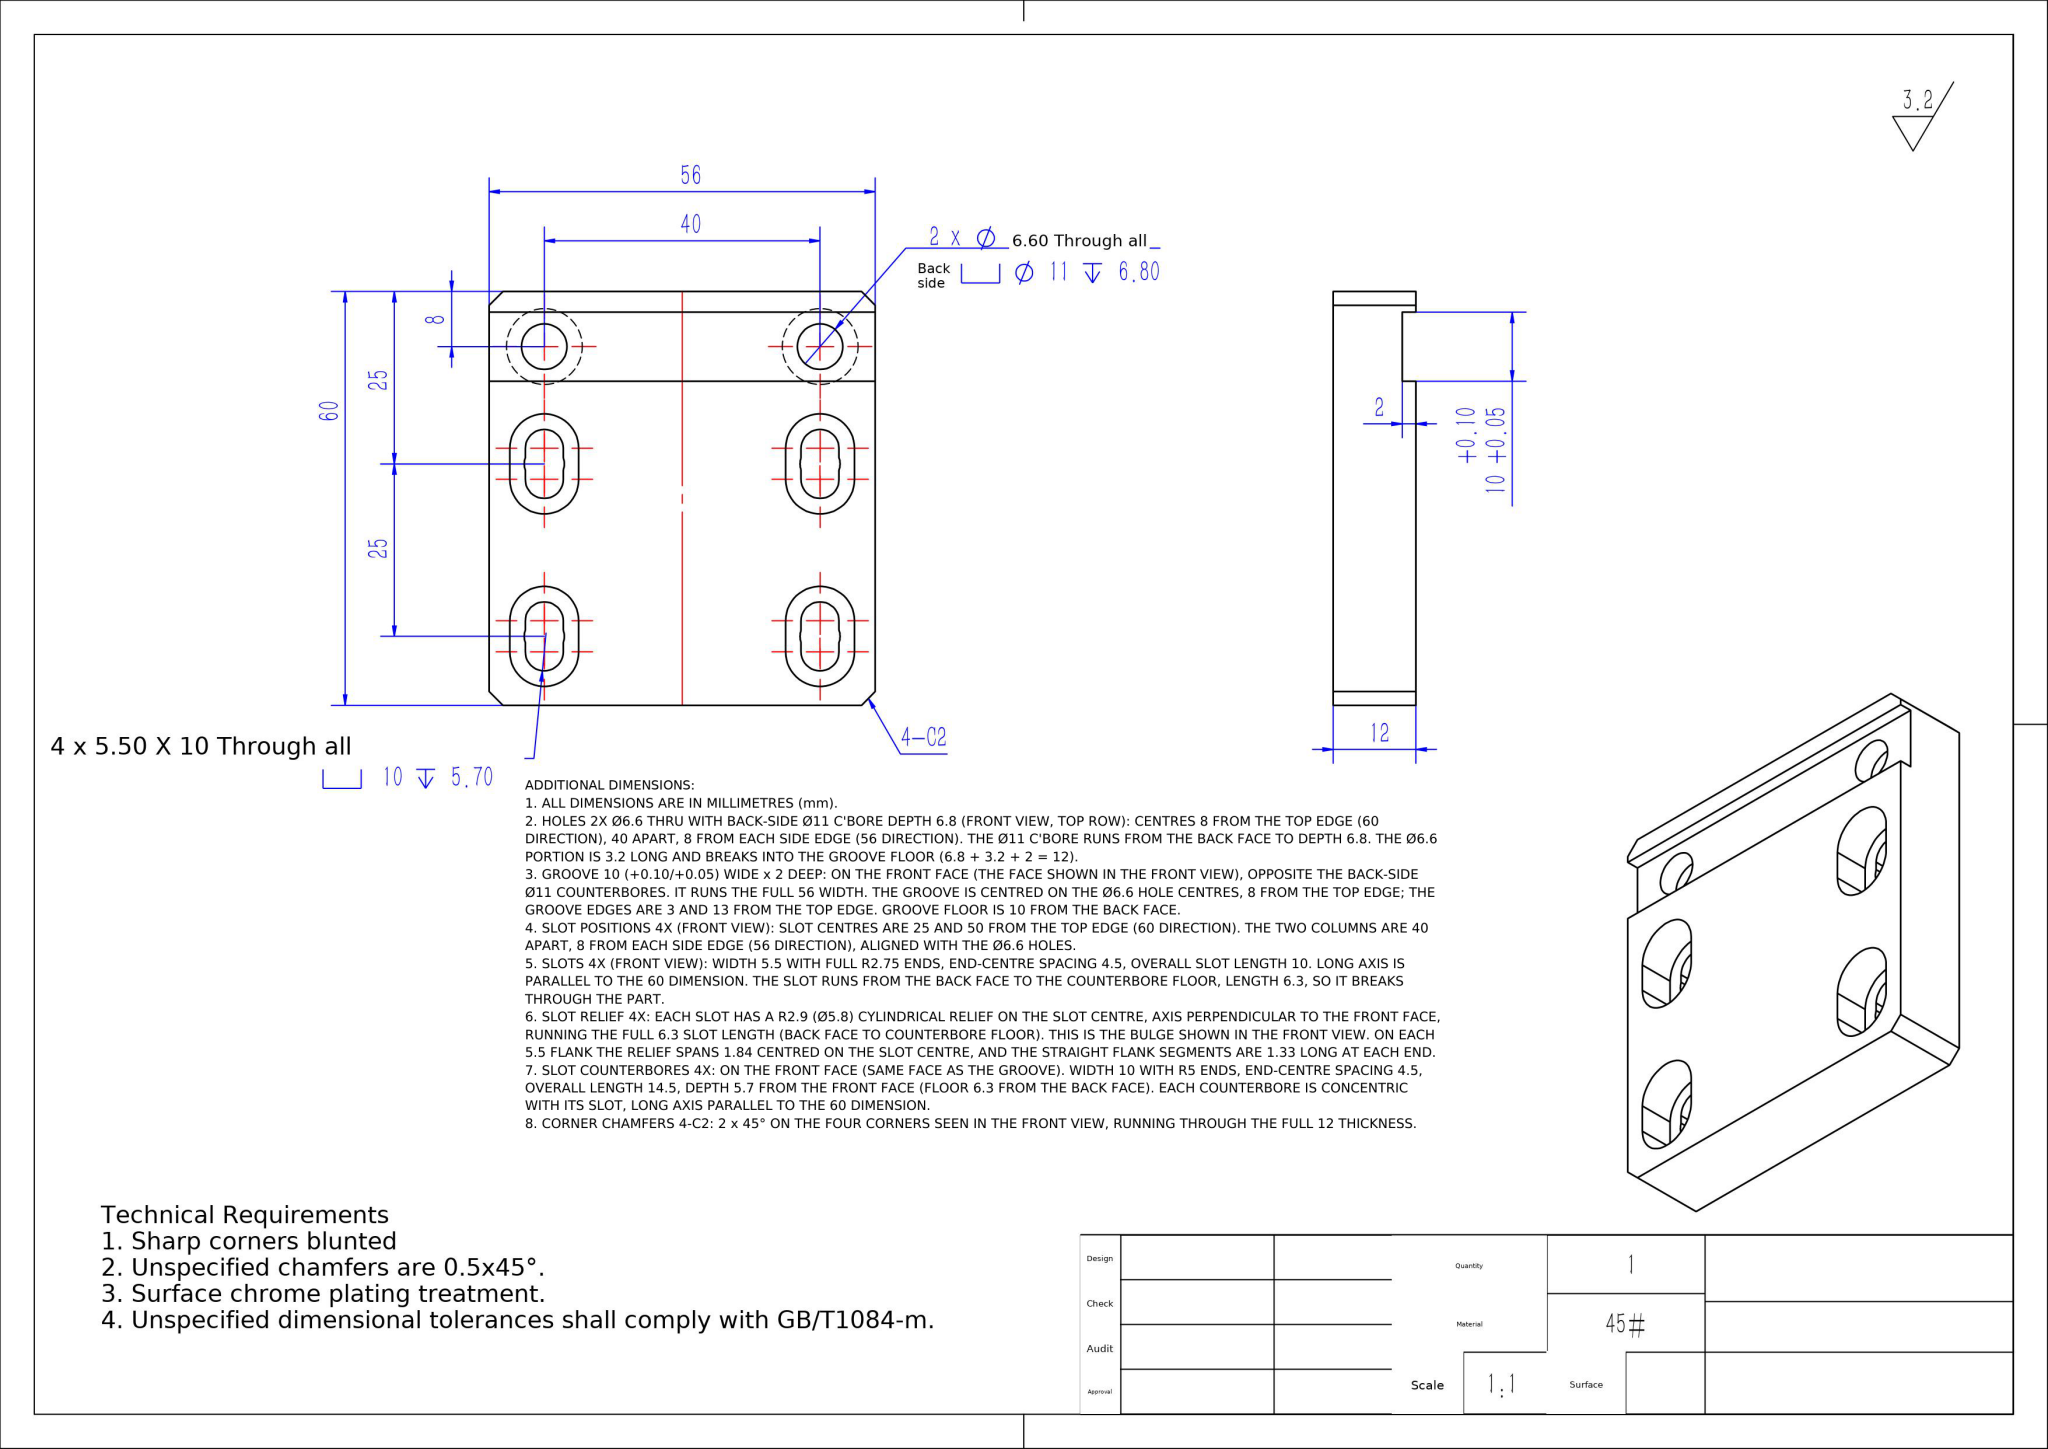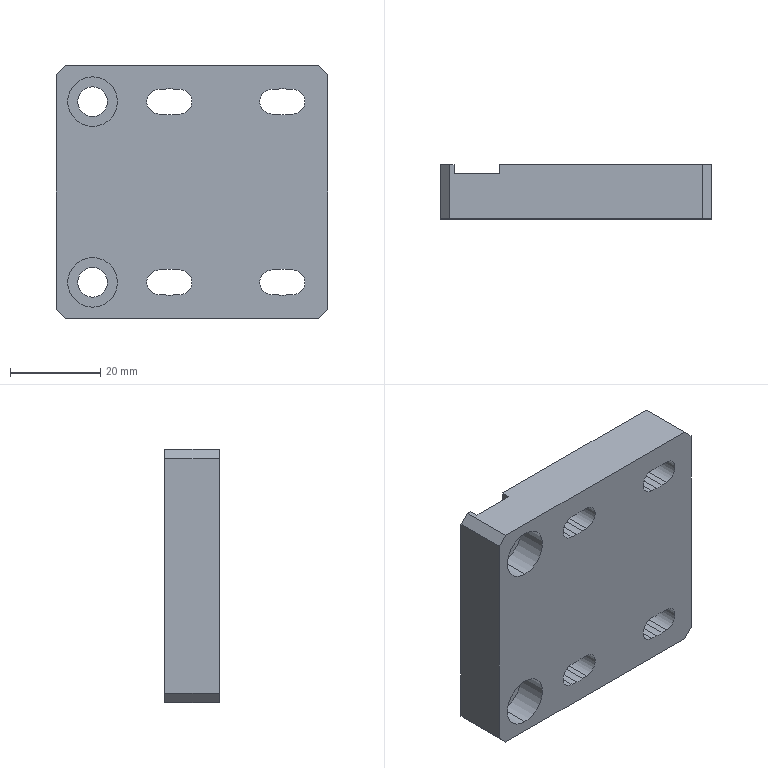Part | NX | mm | 1 solid | 76 faces | box 60 x 12 x 56 mm | volume 33544 mm3 | plane 44 | cylinder 32 | commonest cylinder face diameters 5.5 x8 10 x8 5.8 x8 11 x4 6.6 x4